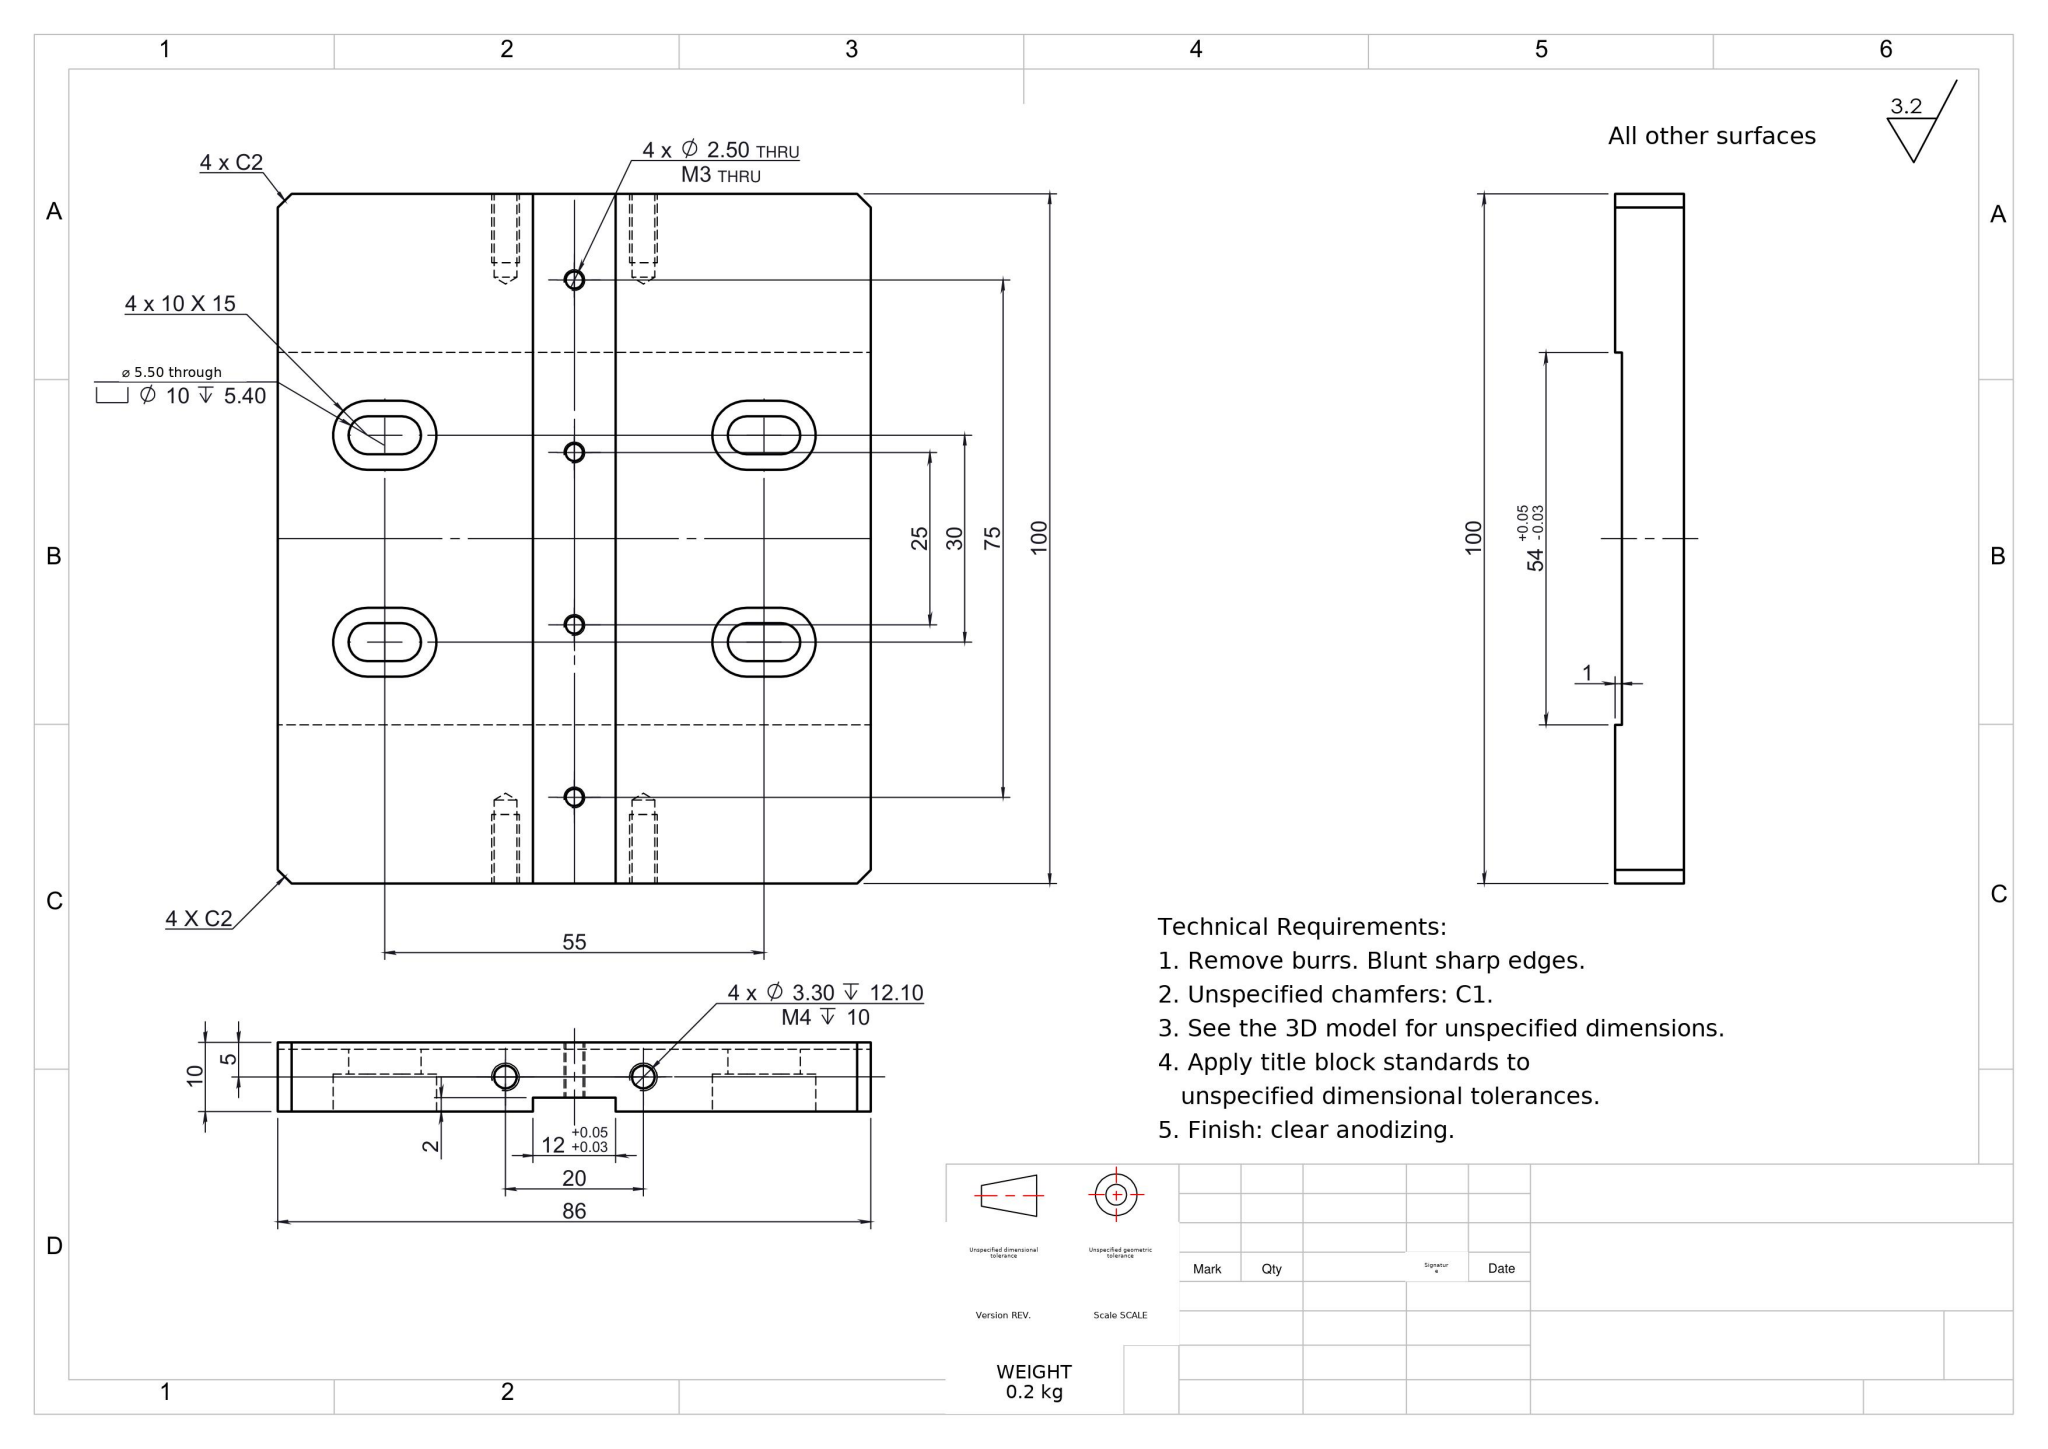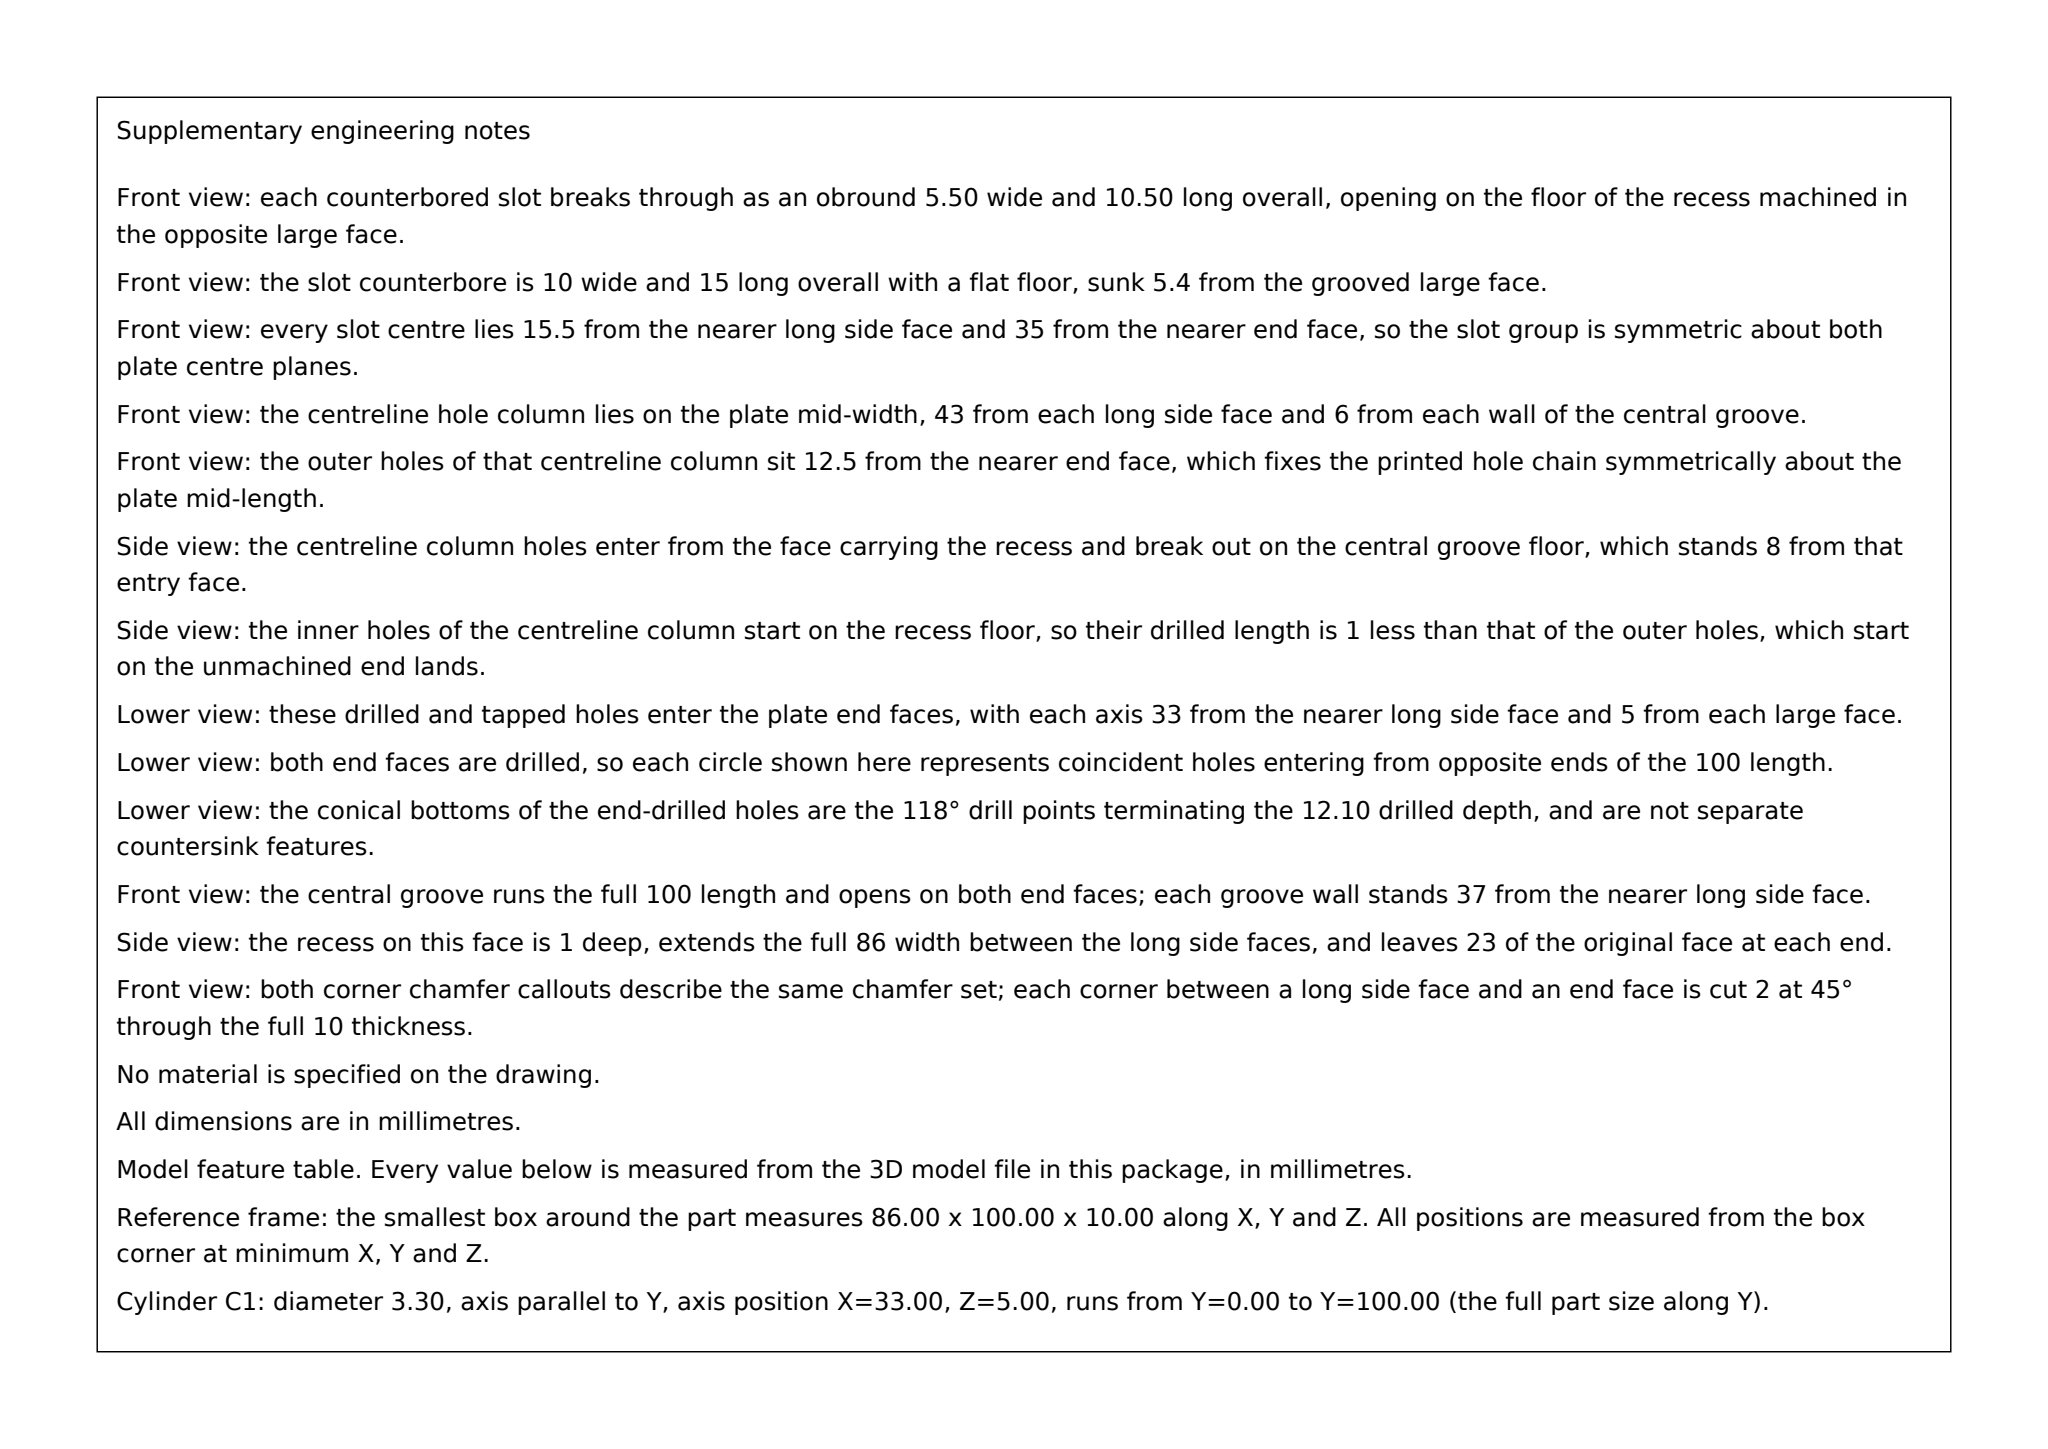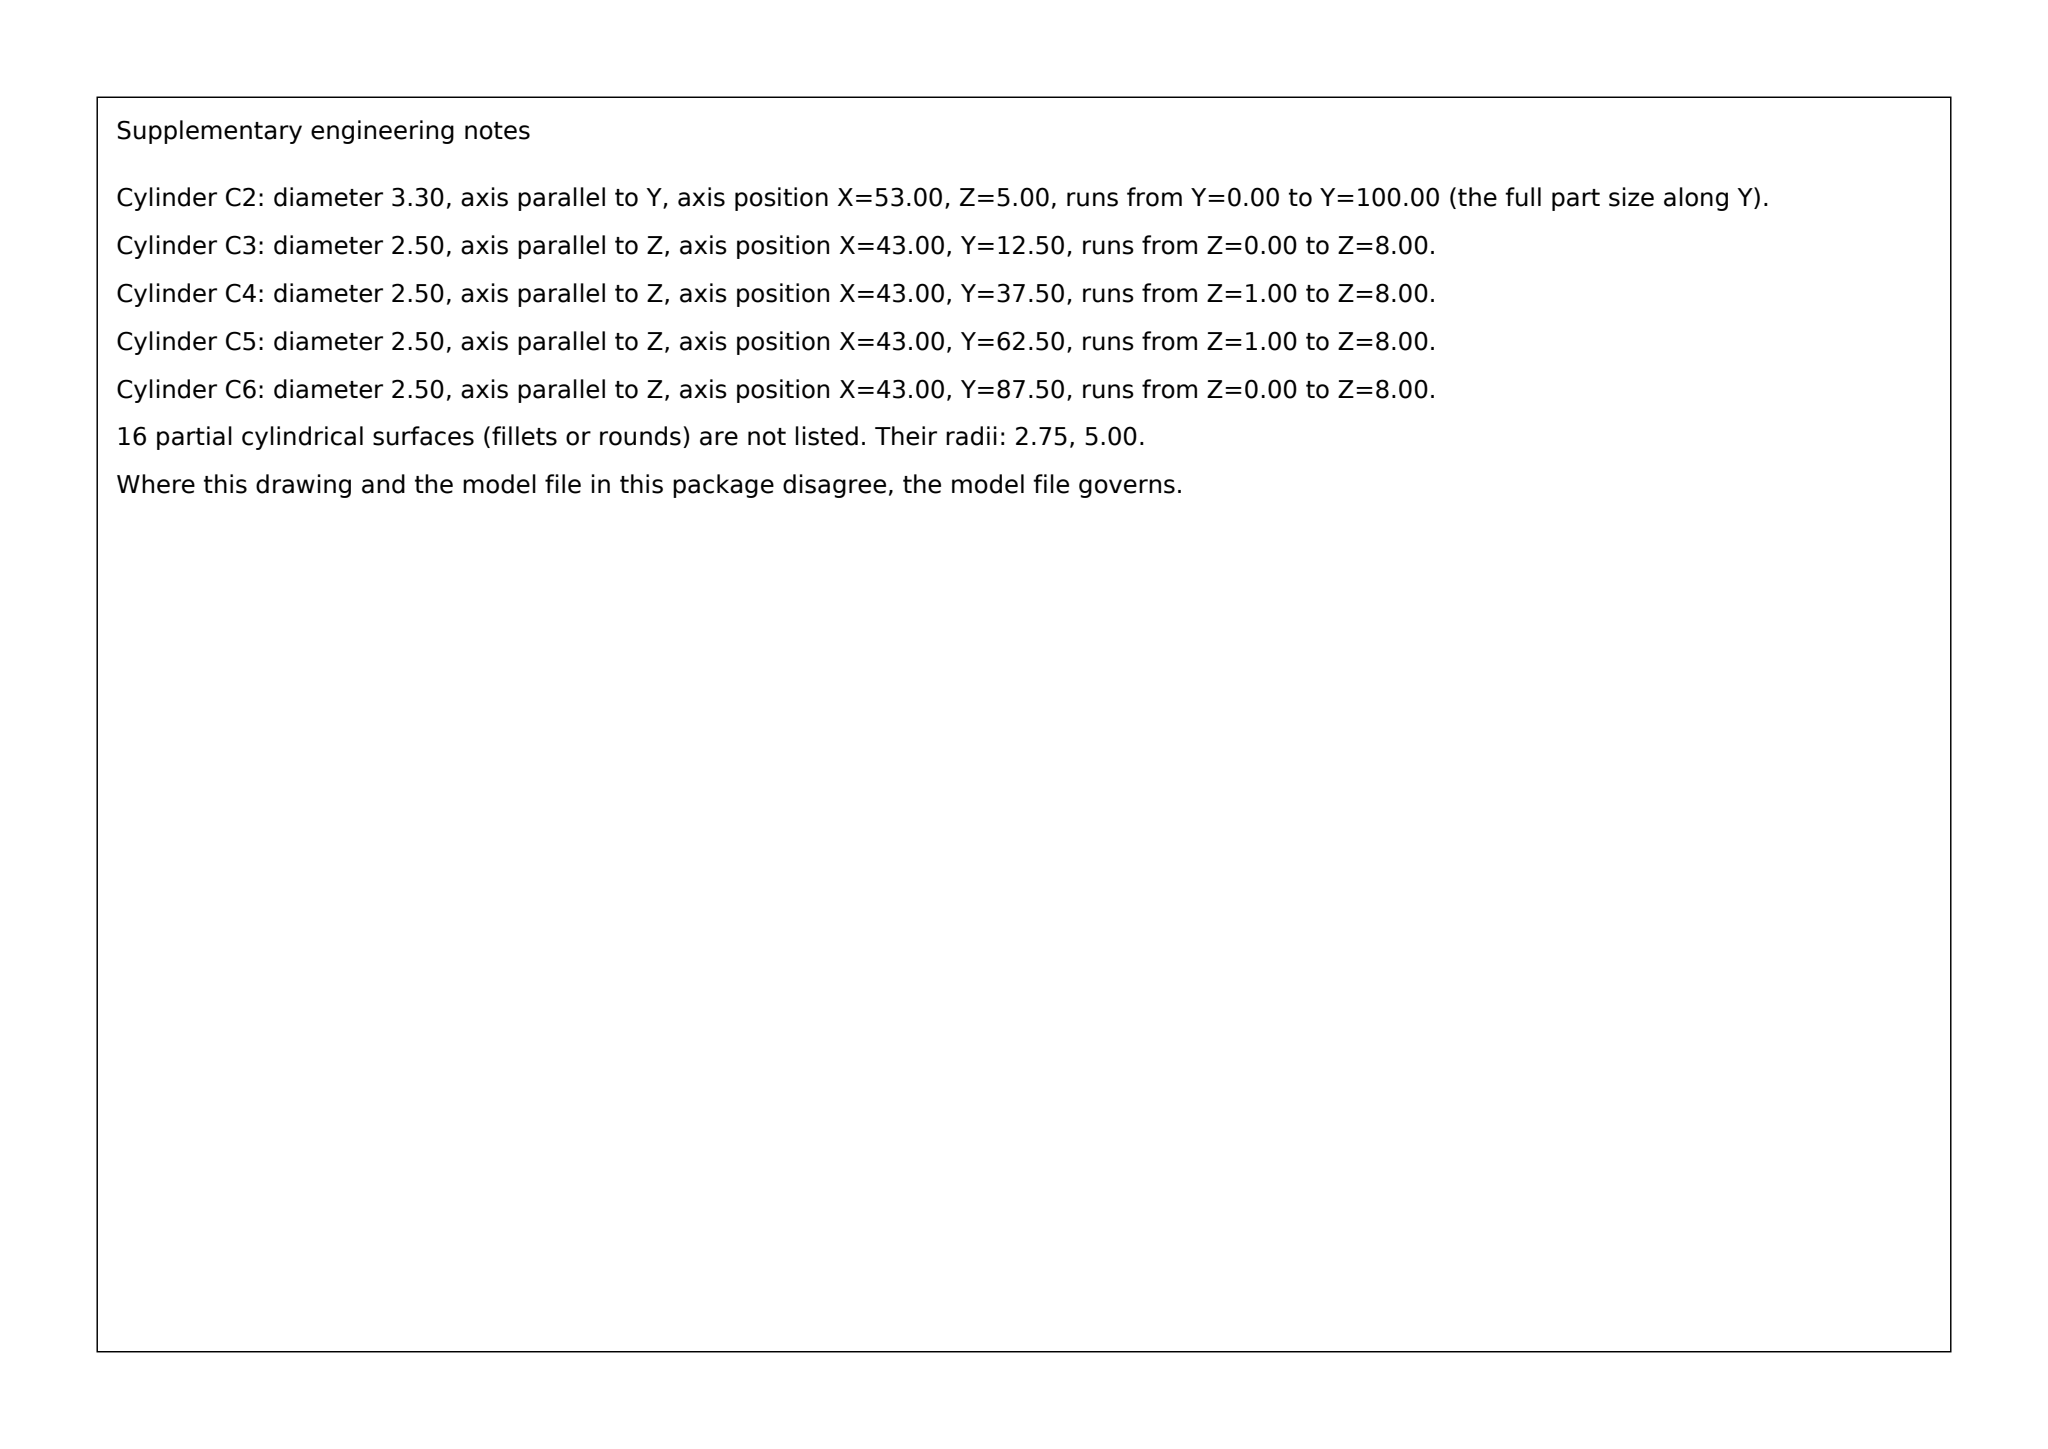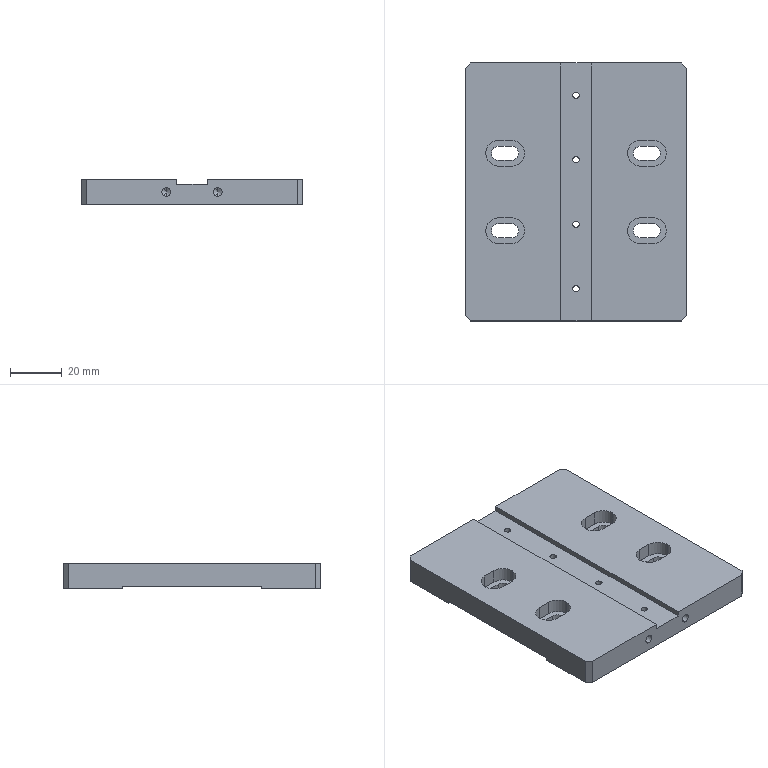Part | SolidWorks | mm | 1 solid | 86 faces | box 86 x 100 x 10 mm | volume 74789 mm3 | cylinder 40 | plane 38 | cone 8 | commonest cylinder face diameters 10 x12 5.5 x12 3.3 x8 2.5 x8
Drawing notes:
4 x Ø2.50 M3 THRU on vert CL, 43 from LH edge | from the solid: cyl Ø2.5 axis z at x=43.0 (bbox X=86)
4 x Ø3.30 DP 12.10 / M4 DP 10: axes 5 from bottom face | from the solid: cyl Ø3.3 axis y at z=5.0, part thk 10 (z 0 to 10)
build123d program:
from build123d import *

# Parameters (mm, degrees)
SKETCH1_W                                       = 86
SKETCH1_H                                       = 100
BOSS_EXTRUDE1_DEPTH                             = 10
SKETCH2_W                                       = 12
SKETCH2_H                                       = 100
CUT_EXTRUDE1_DEPTH                              = 2
M5_HEX_SOCKET_HEAD_CAP_SCREW_CBORE1_D           = 5.5
M5_HEX_SOCKET_HEAD_CAP_SCREW_CBORE1_CBORE_D     = 10
M5_HEX_SOCKET_HEAD_CAP_SCREW_CBORE1_CBORE_DEPTH = 5.4
M3_TAPPED_HOLE1_D                               = 2.5
M4_TAPPED_HOLE1_AT_2_COUNT                      = 2
M4_TAPPED_HOLE1_AT_2_PITCH                      = 20
CHAMFER1_SIZE                                   = 2
SKETCH15_W                                      = 86
SKETCH15_H                                      = 54
CUT_EXTRUDE4_DEPTH                              = 1
CUT_EXTRUDE5_DEPTH                              = 10
CUT_EXTRUDE6_DEPTH                              = 5.4


with BuildPart() as part:
    # Sketch1 → Boss-Extrude1 (new body)
    with BuildSketch(Plane.XY):
        Rectangle(SKETCH1_W, SKETCH1_H)
    extrude(amount=BOSS_EXTRUDE1_DEPTH)

    # Sketch2 → Cut-Extrude1 (cut)
    with BuildSketch(Plane.XY.offset(10)):
        Rectangle(SKETCH2_W, SKETCH2_H)
    extrude(amount=-CUT_EXTRUDE1_DEPTH, mode=Mode.SUBTRACT)

    # M5 Hex Socket Head Cap Screw CBORE1 (through all)
    with Locations(Plane.XY.offset(10)):
        with Locations((-27.5, 15), (27.5, 15), (27.5, -15), (-27.5, -15)):
            CounterBoreHole(M5_HEX_SOCKET_HEAD_CAP_SCREW_CBORE1_D / 2, M5_HEX_SOCKET_HEAD_CAP_SCREW_CBORE1_CBORE_D / 2, M5_HEX_SOCKET_HEAD_CAP_SCREW_CBORE1_CBORE_DEPTH)

    # M3 Tapped Hole1 (through all)
    with Locations(Plane.XY.offset(8)):
        with Locations((0, -37.5), (0, -12.5), (0, 12.5), (0, 37.5)):
            Hole(M3_TAPPED_HOLE1_D / 2)

    # Sketch8 → M4 Tapped Hole1 (revolve, cut)
    with BuildSketch(Plane(origin=(-10, 50, 5), x_dir=(0, 0, 1), z_dir=(1, 0, 0))):
        Polygon((0, 0), (0, 13.091), (1.65, 12.1), (1.65, 0), align=None)
    m4_tapped_hole1 = revolve(axis=Axis((-10, 56.35, 5), (0, -1, 0)), mode=Mode.SUBTRACT)

    # M4 Tapped Hole1 at 2: M4 Tapped Hole1 ×2
    with Locations(*[(i * M4_TAPPED_HOLE1_AT_2_PITCH, 0, 0) for i in range(1, M4_TAPPED_HOLE1_AT_2_COUNT)]):
        add(m4_tapped_hole1, mode=Mode.SUBTRACT)

    # Mirror1: M4 Tapped Hole1 across plane
    add(m4_tapped_hole1.mirror(Plane.ZX), mode=Mode.SUBTRACT)

    # Mirror1 copy 1 sketch → Mirror1 copy 1 (revolve, cut)
    with BuildSketch(Plane(origin=(10, -50, 5), x_dir=(0, 0, 1), z_dir=(1, 0, 0))):
        Polygon((0, 0), (0, -13.091), (1.65, -12.1), (1.65, 0), align=None)
    revolve(axis=Axis((10, -56.35, 5), (0, -1, 0)), mode=Mode.SUBTRACT)

    # Chamfer1
    chamfer1_edges = [part.edges().sort_by_distance(p)[0] for p in [
        (-43, 50, 5),
        (43, 50, 5),
        (43, -50, 5),
        (-43, -50, 5),
    ]]
    chamfer(chamfer1_edges, length=CHAMFER1_SIZE)

    # Sketch15 → Cut-Extrude4 (cut)
    with BuildSketch(Plane(origin=(0, 0, 0), x_dir=(-1, 0, 0), z_dir=(0, 0, -1))):
        Rectangle(SKETCH15_W, SKETCH15_H)
    extrude(amount=-CUT_EXTRUDE4_DEPTH, mode=Mode.SUBTRACT)

    # Sketch19 → Cut-Extrude5 (cut)
    with BuildSketch(Plane.XY.offset(10)):
        with BuildLine():
            Line((-30, -12.25), (-25, -12.25))
            ThreePointArc((-25, -12.25), (-22.25, -15), (-25, -17.75))
            Line((-25, -17.75), (-30, -17.75))
            ThreePointArc((-30, -17.75), (-32.75, -15), (-30, -12.25))
        make_face()
        with BuildLine():
            Line((-30, 12.25), (-25, 12.25))
            ThreePointArc((-25, 12.25), (-22.25, 15), (-25, 17.75))
            Line((-25, 17.75), (-30, 17.75))
            ThreePointArc((-30, 17.75), (-32.75, 15), (-30, 12.25))
        make_face()
        with BuildLine():
            Line((30, 12.25), (25, 12.25))
            ThreePointArc((25, 12.25), (22.25, 15), (25, 17.75))
            Line((25, 17.75), (30, 17.75))
            ThreePointArc((30, 17.75), (32.75, 15), (30, 12.25))
        make_face()
        with BuildLine():
            Line((30, -12.25), (25, -12.25))
            ThreePointArc((25, -12.25), (22.25, -15), (25, -17.75))
            Line((25, -17.75), (30, -17.75))
            ThreePointArc((30, -17.75), (32.75, -15), (30, -12.25))
        make_face()
    extrude(amount=-CUT_EXTRUDE5_DEPTH, mode=Mode.SUBTRACT)

    # Sketch20 → Cut-Extrude6 (cut)
    with BuildSketch(Plane.XY.offset(10)):
        with BuildLine():
            Line((-30, -10), (-25, -10))
            ThreePointArc((-25, -10), (-20, -15), (-25, -20))
            Line((-25, -20), (-30, -20))
            ThreePointArc((-30, -20), (-35, -15), (-30, -10))
        make_face()
        with BuildLine():
            Line((-30, 10), (-25, 10))
            ThreePointArc((-25, 10), (-20, 15), (-25, 20))
            Line((-25, 20), (-30, 20))
            ThreePointArc((-30, 20), (-35, 15), (-30, 10))
        make_face()
        with BuildLine():
            Line((30, 10), (25, 10))
            ThreePointArc((25, 10), (20, 15), (25, 20))
            Line((25, 20), (30, 20))
            ThreePointArc((30, 20), (35, 15), (30, 10))
        make_face()
        with BuildLine():
            Line((30, -10), (25, -10))
            ThreePointArc((25, -10), (20, -15), (25, -20))
            Line((25, -20), (30, -20))
            ThreePointArc((30, -20), (35, -15), (30, -10))
        make_face()
    extrude(amount=-CUT_EXTRUDE6_DEPTH, mode=Mode.SUBTRACT)


solid = part.part